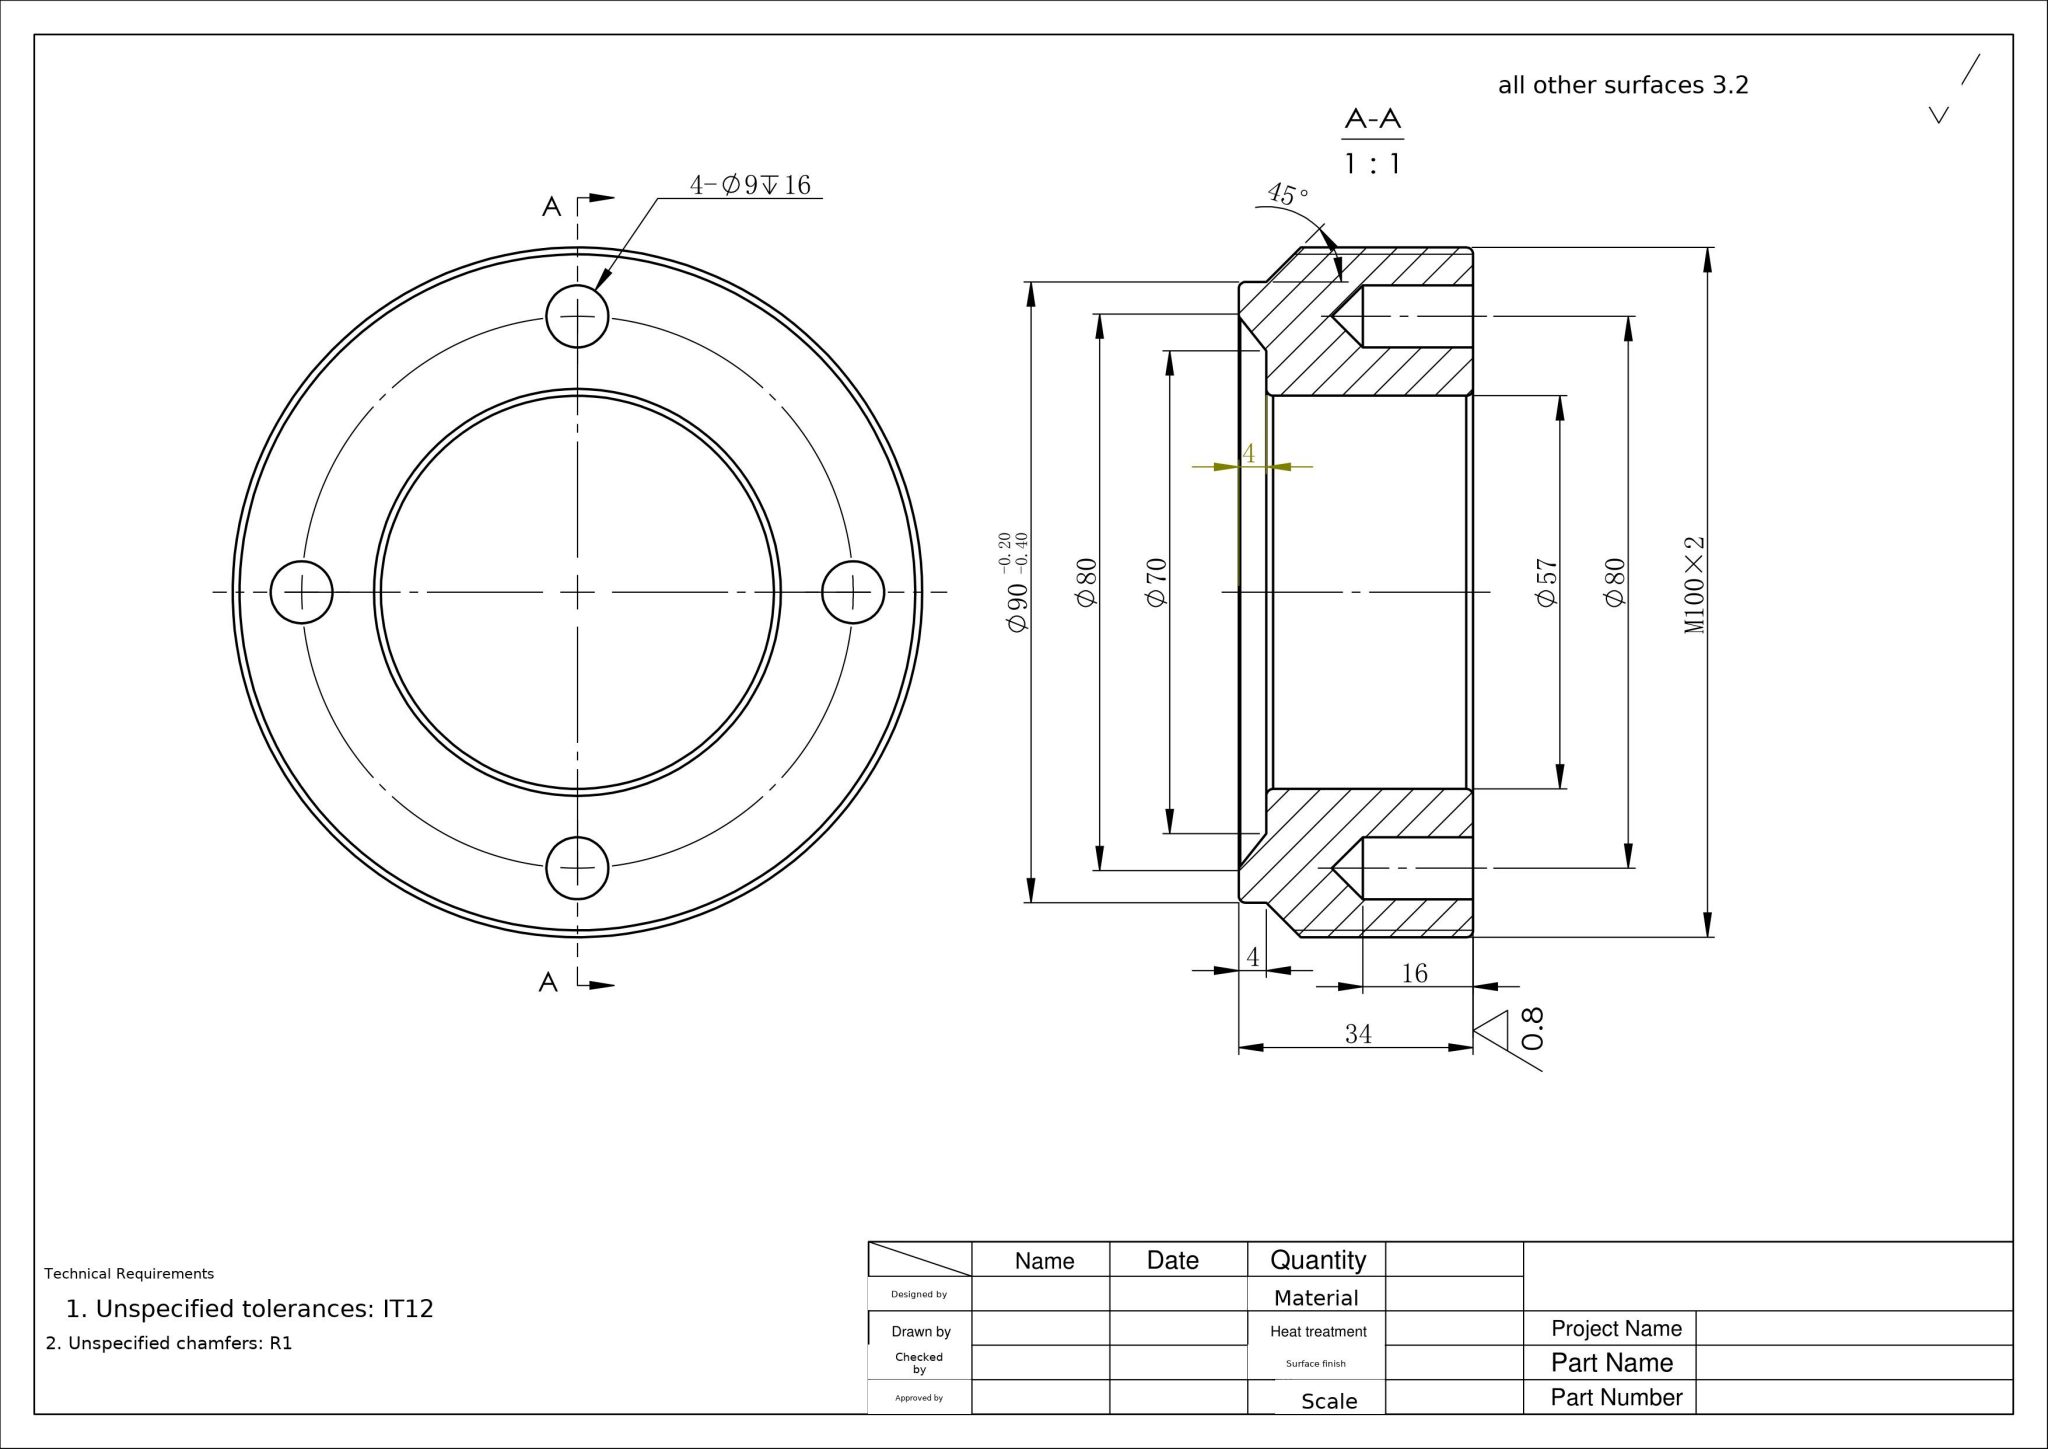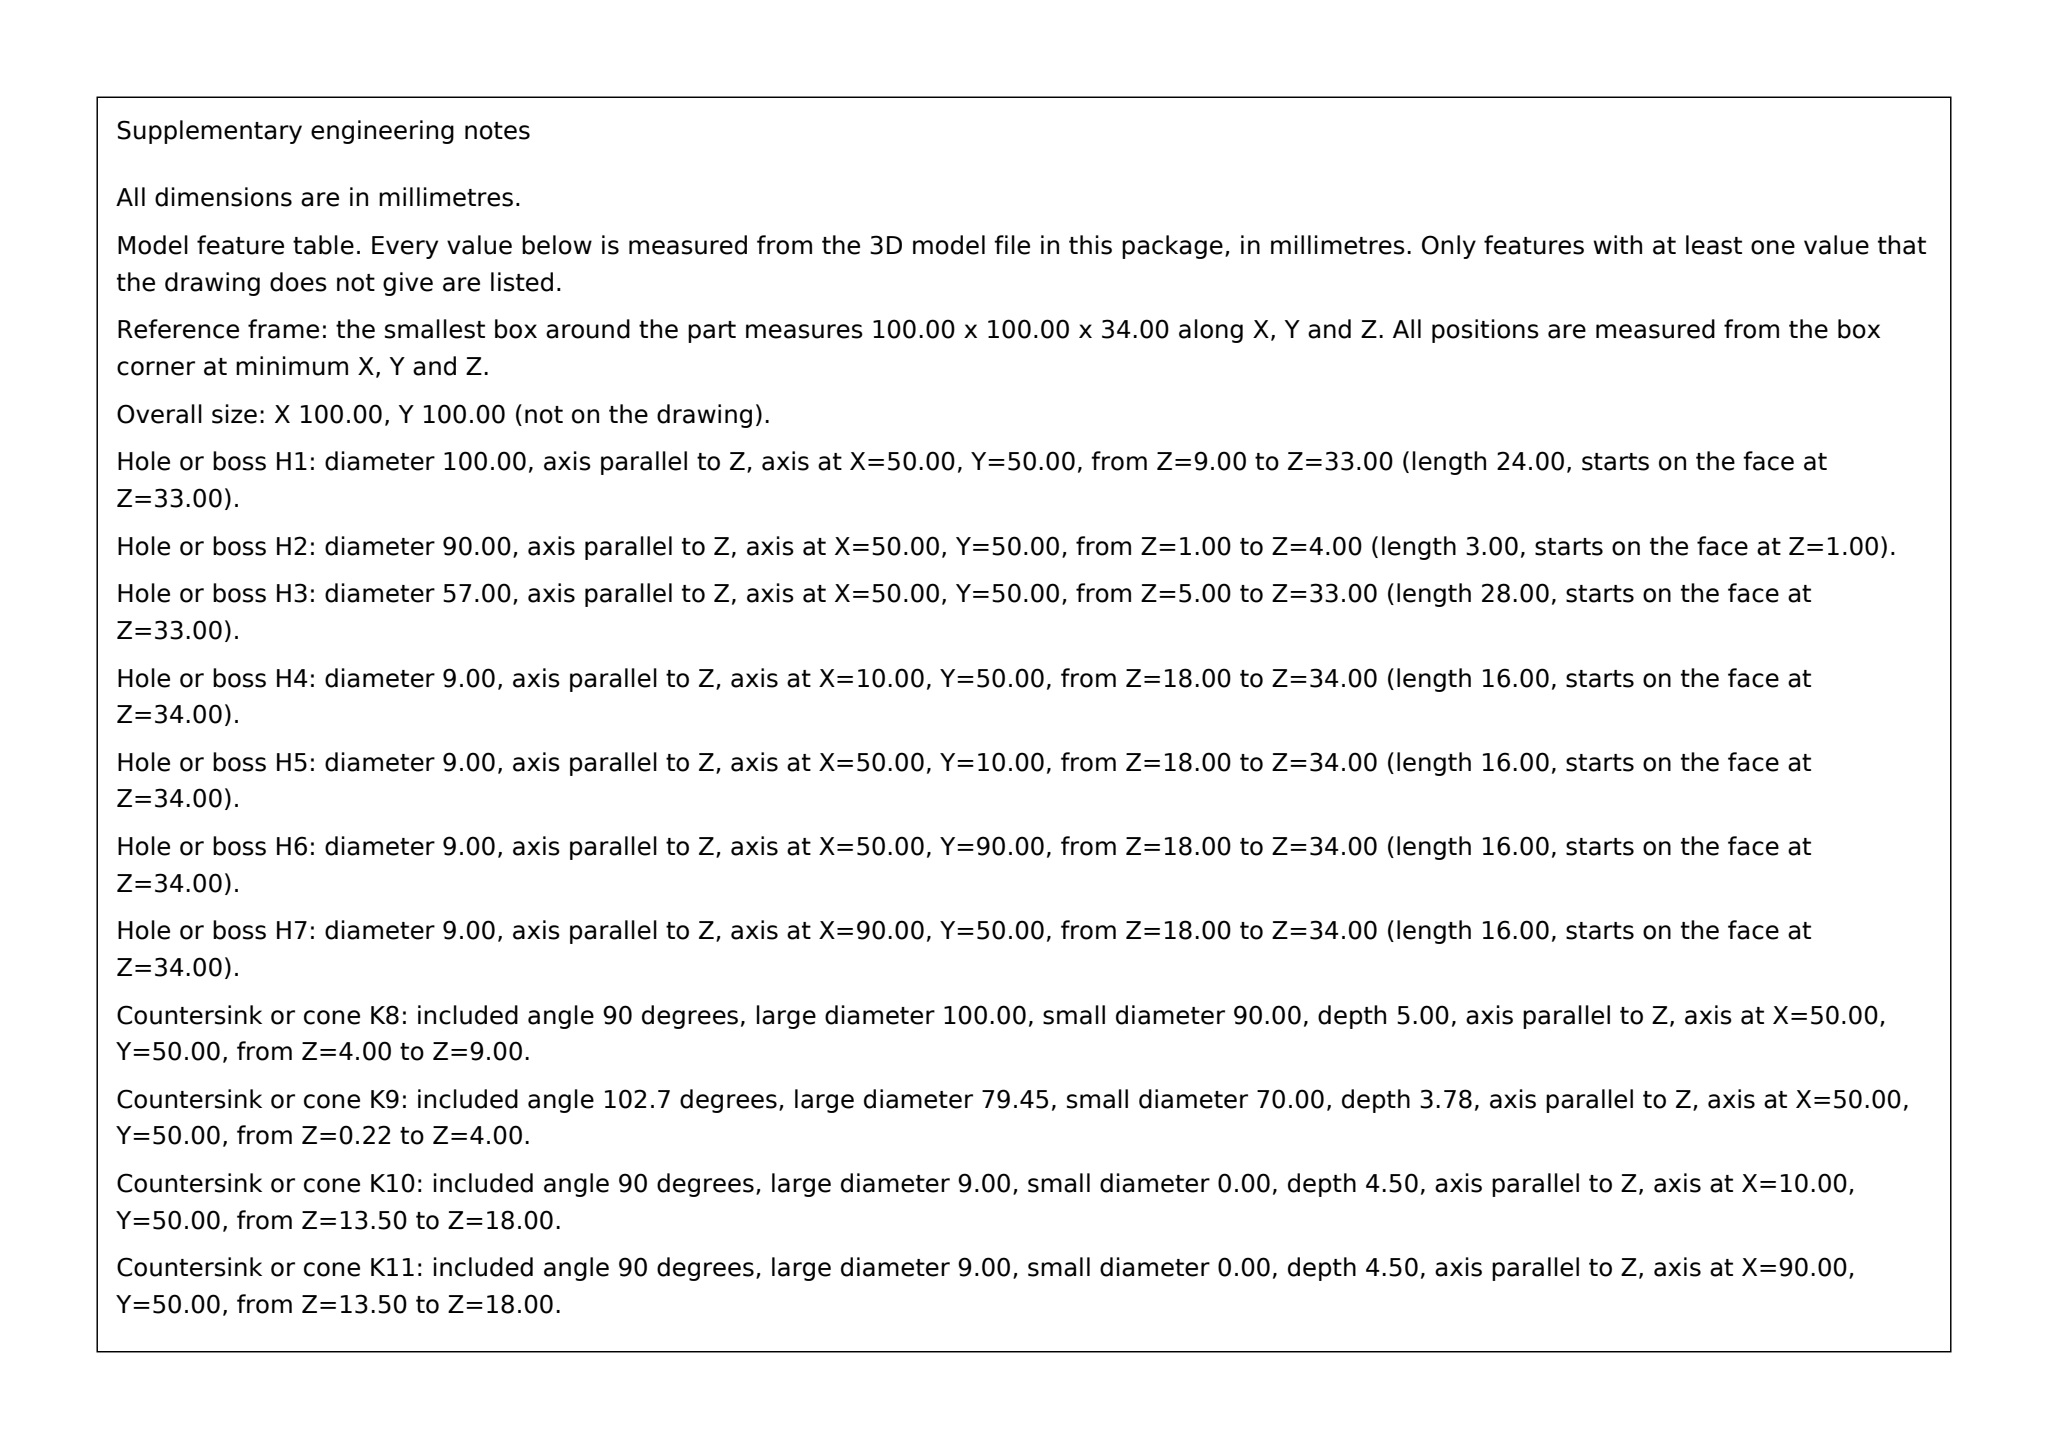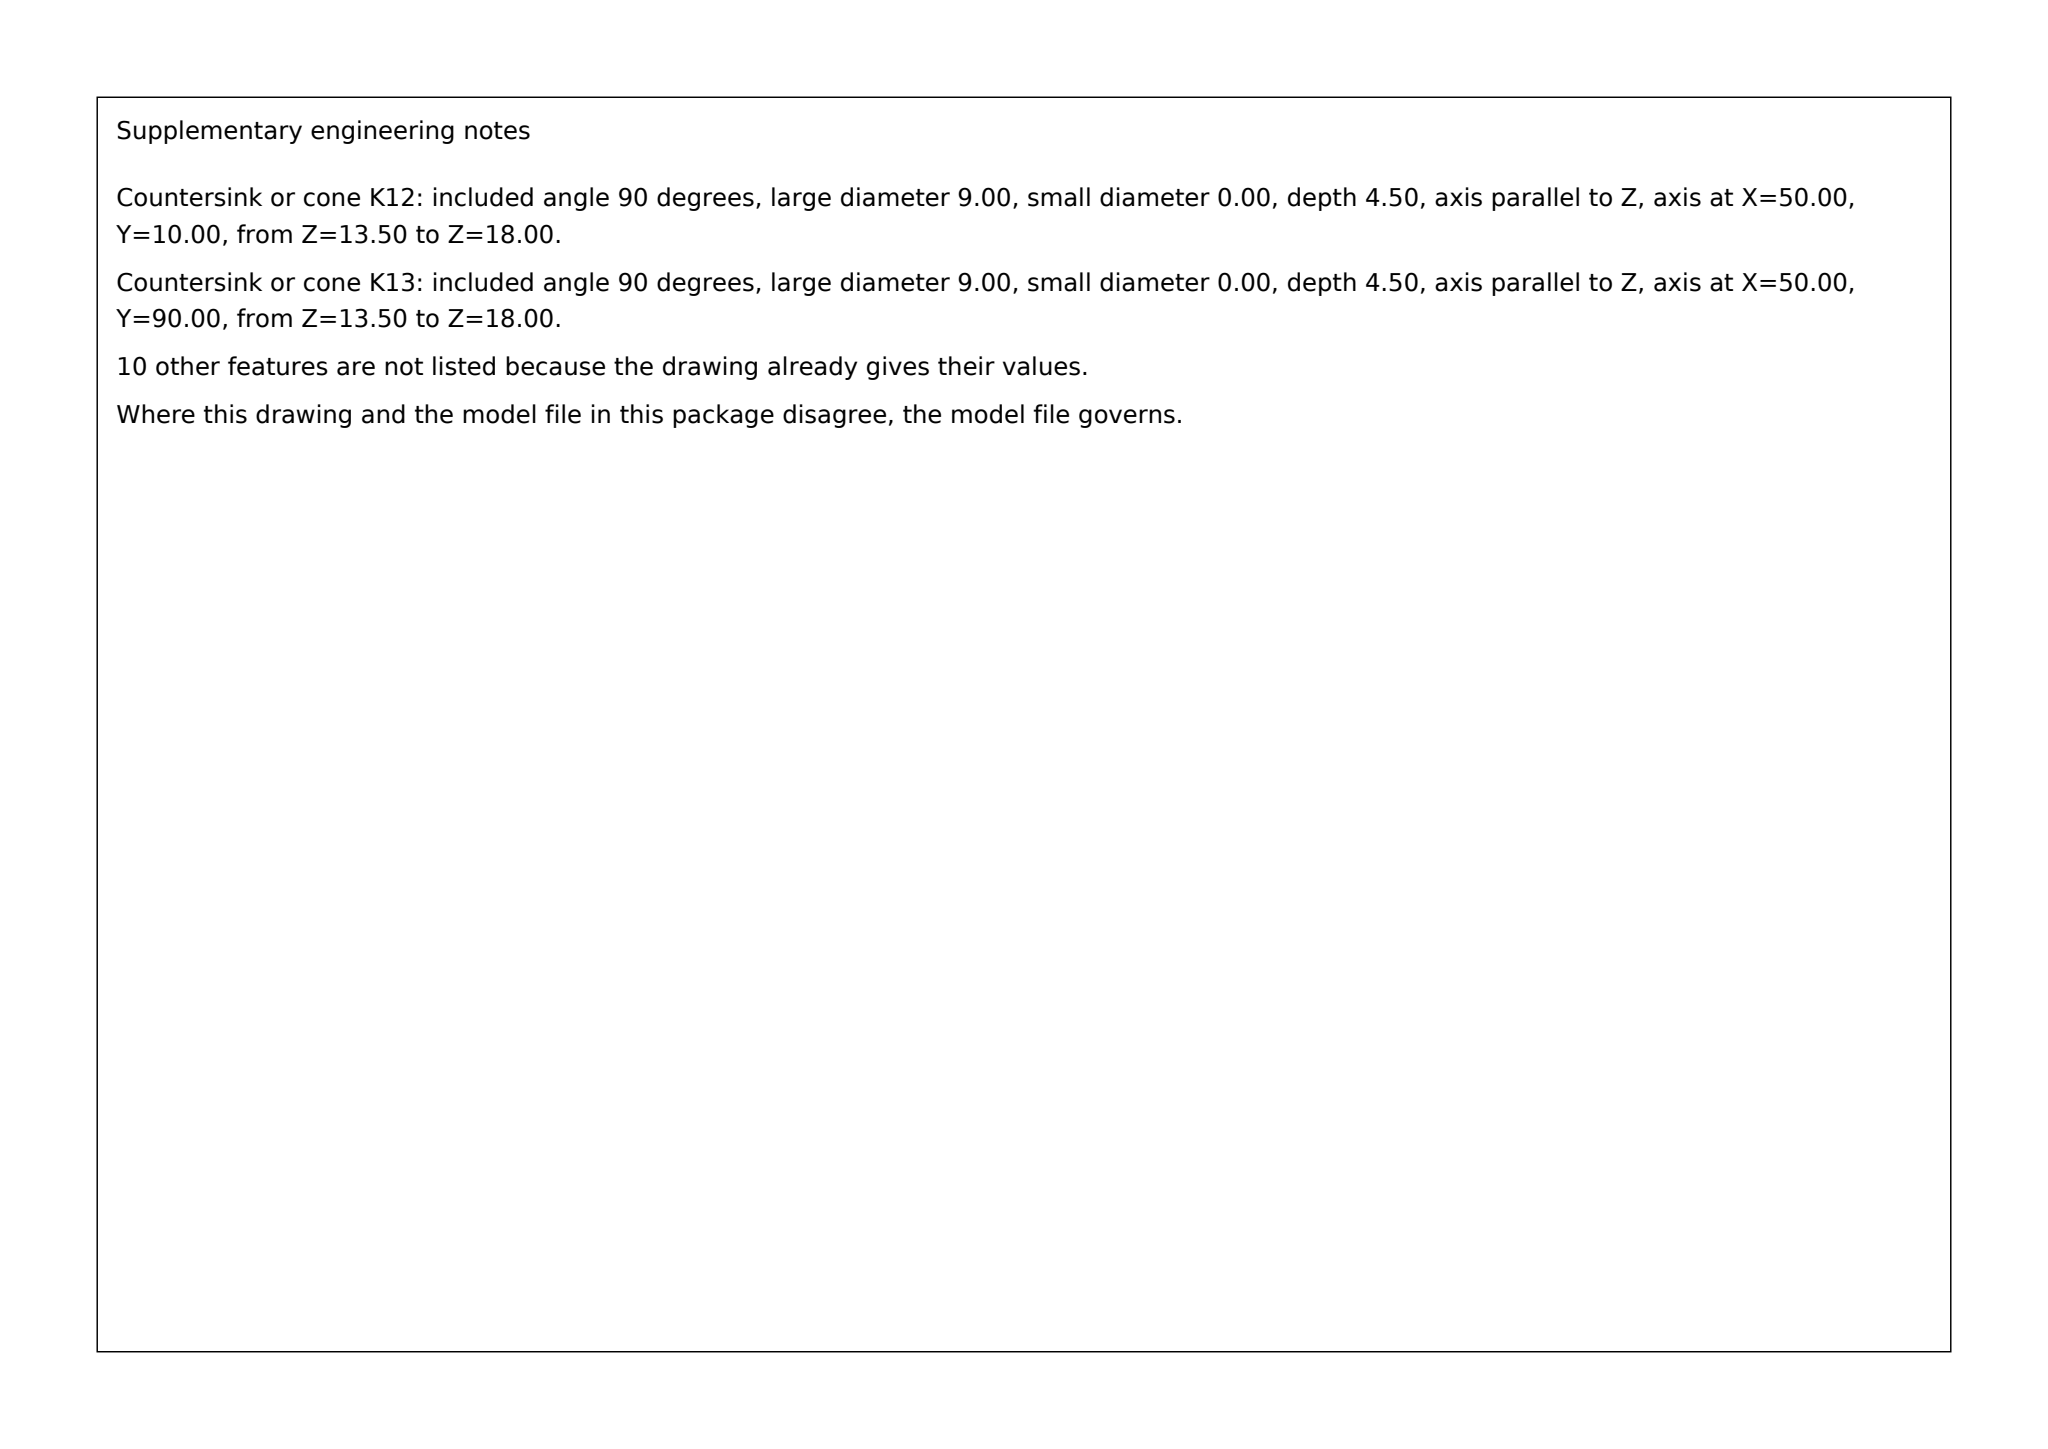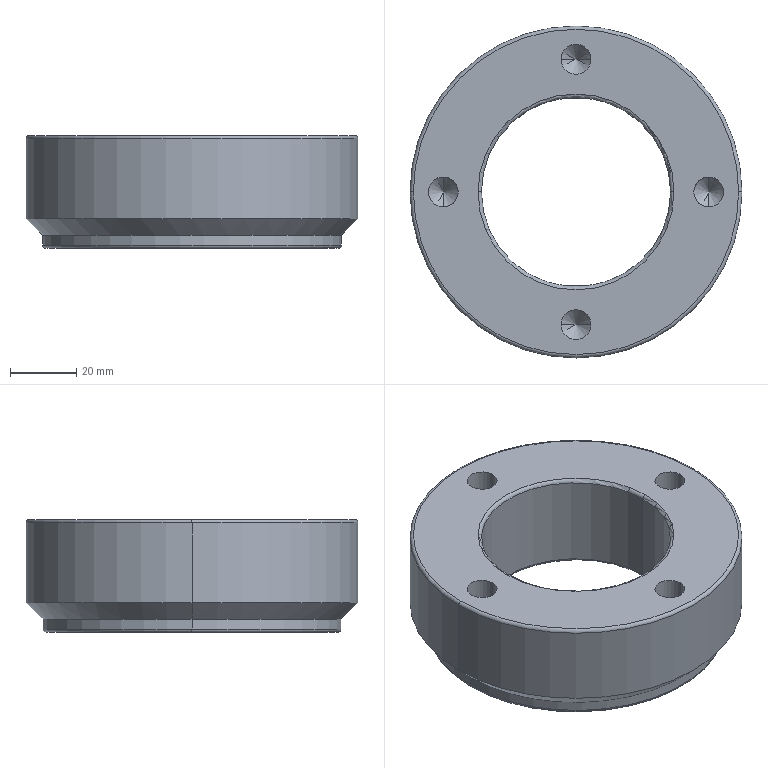Part | SolidWorks | mm | 1 solid | 39 faces | box 100 x 100 x 34 mm | volume 158358 mm3 | cylinder 14 | cone 12 | torus 10 | plane 3 | commonest cylinder face diameters 9 x8 90 x2 100 x2 57 x2
build123d program:
from build123d import *

# Parameters (mm, degrees)
SKETCH1_R          = 50
EXTRUDE1_DEPTH     = 34
SKETCH2_R          = 28.5
CUT_EXTRUDE1_DEPTH = 79.46
SKETCH3_R          = 57.174
SKETCH3_R_2        = 45
CUT_EXTRUDE2_DEPTH = 4
SKETCH4_R          = 35
CUT_EXTRUDE3_DEPTH = 4
SKETCH8_R          = 4.5
CUT_EXTRUDE4_DEPTH = 16
CIRPATTERN1_COUNT  = 4
FILLET1_R          = 1


with BuildPart() as part:
    # Sketch1 → Extrude1 (new body)
    with BuildSketch(Plane.XY):
        Circle(SKETCH1_R)
    extrude(amount=EXTRUDE1_DEPTH)

    # Sketch2 → Cut-Extrude1 (cut, through all)
    with BuildSketch(Plane(origin=(0, 0, 0), x_dir=(-1, 0, 0), z_dir=(0, 0, -1))):
        Circle(SKETCH2_R)
    extrude(amount=-CUT_EXTRUDE1_DEPTH, mode=Mode.SUBTRACT)

    # Sketch3 → Cut-Extrude2 (cut)
    with BuildSketch(Plane(origin=(0, 0, 0), x_dir=(-1, 0, 0), z_dir=(0, 0, -1))):
        Circle(SKETCH3_R)
        Circle(SKETCH3_R_2, mode=Mode.SUBTRACT)
    extrude(amount=-CUT_EXTRUDE2_DEPTH, mode=Mode.SUBTRACT)

    # Sketch4 → Cut-Extrude3 (cut)
    with BuildSketch(Plane(origin=(0, 0, 0), x_dir=(-1, 0, 0), z_dir=(0, 0, -1))):
        Circle(SKETCH4_R)
    extrude(amount=-CUT_EXTRUDE3_DEPTH, mode=Mode.SUBTRACT)

    # Sketch5 → Cut-Revolve1 (revolve, cut)
    with BuildSketch(Plane(origin=(0, 0, 0), x_dir=(1, 0, 0), z_dir=(0, 1, 0))):
        Polygon((-35, -4), (-40, 0), (-35, 0), align=None)
        Polygon((-45, -4), (-50, -9), (-50, -4), align=None)
    revolve(axis=Axis((0, 0, 0), (0, 0, 1)), mode=Mode.SUBTRACT)

    # Sketch8 → Cut-Extrude4 (cut)
    with BuildSketch(Plane.XY.offset(34)):
        with Locations((0, 40)):
            Circle(SKETCH8_R)
    cut_extrude4 = extrude(amount=-CUT_EXTRUDE4_DEPTH, mode=Mode.SUBTRACT)

    # Sketch9 → Cut-Revolve2 (revolve, cut)
    with BuildSketch(Plane(origin=(0, 0, 0), x_dir=(0, 0, -1), z_dir=(1, 0, 0)), mode=Mode.PRIVATE) as cut_revolve2_sk:
        Polygon((-18, 44.5), (-13.5, 40), (-18, 40), align=None)
    cut_revolve2 = revolve(cut_revolve2_sk.sketch.rotate(Axis((0, 40, 38.27), (0, 0, -1)), 90), axis=Axis((0, 40, 38.27), (0, 0, -1)), mode=Mode.SUBTRACT)

    # CirPattern1: Cut-Extrude4, Cut-Revolve2 ×4 about axis
    cirpattern1_axis = Axis((0, 0, 0), (0, 0, 1))
    add([cut_extrude4.rotate(cirpattern1_axis, i * 360 / CIRPATTERN1_COUNT) for i in range(1, CIRPATTERN1_COUNT)], mode=Mode.SUBTRACT)
    add([cut_revolve2.rotate(cirpattern1_axis, i * 360 / CIRPATTERN1_COUNT) for i in range(1, CIRPATTERN1_COUNT)], mode=Mode.SUBTRACT)

    # Fillet1
    fillet1_edges = [part.edges().sort_by_distance(p)[0] for p in [
        (45, 0, 0),
        (28.5, 0, 4),
        (40, 0, 0),
        (-50, 0, 34),
        (28.5, 0, 34),
    ]]
    fillet(fillet1_edges, radius=FILLET1_R)


solid = part.part